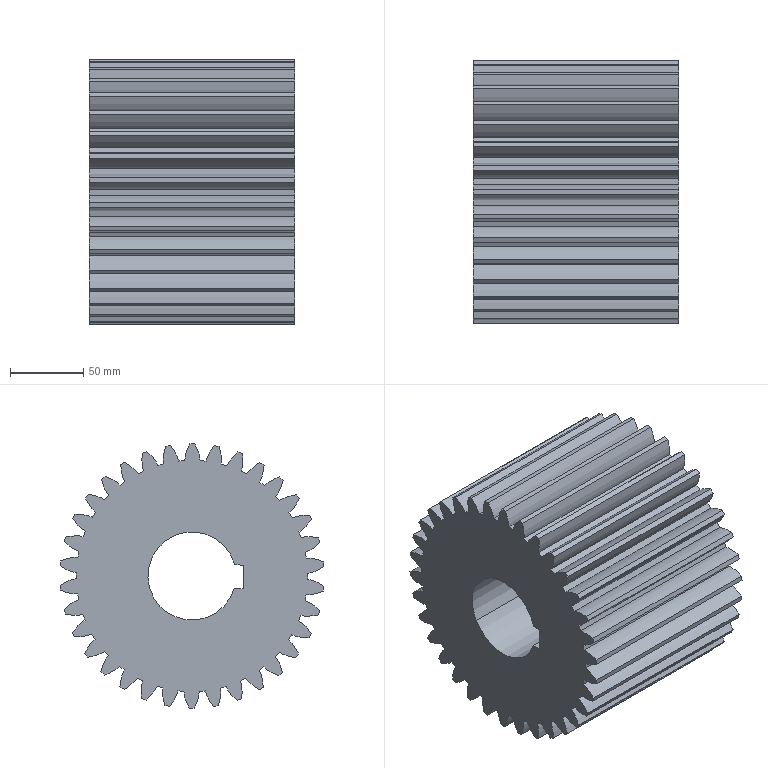Component | SolidWorks | Pinion-1 | 1 solid | 144 faces | box 140 x 179.55 x 179.98 mm | volume 2739604 mm3 | plane 73 | spline 68 | cylinder 3 | commonest cylinder face diameters 60 x3
build123d program:
from build123d import *

# Parameters (mm, degrees)
BOSS_EXTRUDE1_DEPTH           = 140
SKETCH1_R                     = 30
REPAIR_BORETOSHAFTDIA60_DEPTH = 71.5


with BuildPart() as part:
    # Sketch1_2 → Boss-Extrude1 (new body)
    with BuildSketch(Plane.XY.offset(140)):
        with BuildLine():
            Line((78.053, 10.453), (77.409, 14.47))
            add(Edge.make_bspline(
                [(77.409, 14.47), (82.062, 15.66), (87.574, 20.756)],
                knots=[3.749, 3.749, 3.749, 4.922, 4.922, 4.922], degree=2, weights=[1, 0.8327, 1]))
            Line((87.574, 20.756), (86.739, 24.006))
            add(Edge.make_bspline(
                [(86.739, 24.006), (79.432, 25.831), (74.803, 24.617)],
                knots=[1.318, 1.318, 1.318, 2.544, 2.544, 2.544], degree=2, weights=[1, 0.8179, 1]))
            Line((74.803, 24.617), (73.432, 28.448))
            add(Edge.make_bspline(
                [(73.432, 28.448), (77.787, 30.472), (82.269, 36.495)],
                knots=[0.607, 0.607, 0.607, 1.781, 1.781, 1.781], degree=2, weights=[1, 0.8327, 1]))
            Line((82.269, 36.495), (80.851, 39.536))
            add(Edge.make_bspline(
                [(80.851, 39.536), (73.333, 39.987), (69.006, 37.943)],
                knots=[1.318, 1.318, 1.318, 2.544, 2.544, 2.544], degree=2, weights=[1, 0.8179, 1]))
            Line((69.006, 37.943), (66.955, 41.457))
            add(Edge.make_bspline(
                [(66.955, 41.457), (70.864, 44.247), (74.162, 50.99)],
                knots=[0.607, 0.607, 0.607, 1.781, 1.781, 1.781], degree=2, weights=[1, 0.8327, 1]))
            Line((74.162, 50.99), (72.21, 53.719))
            add(Edge.make_bspline(
                [(72.21, 53.719), (64.737, 52.781), (60.859, 49.977)],
                knots=[1.318, 1.318, 1.318, 2.544, 2.544, 2.544], degree=2, weights=[1, 0.8179, 1]))
            Line((60.859, 49.977), (58.197, 53.054))
            add(Edge.make_bspline(
                [(58.197, 53.054), (61.527, 56.514), (63.53, 63.749)],
                knots=[0.607, 0.607, 0.607, 1.781, 1.781, 1.781], degree=2, weights=[1, 0.8327, 1]))
            Line((63.53, 63.749), (61.109, 66.073))
            add(Edge.make_bspline(
                [(61.109, 66.073), (53.936, 63.777), (50.64, 60.309)],
                knots=[1.318, 1.318, 1.318, 2.544, 2.544, 2.544], degree=2, weights=[1, 0.8179, 1]))
            Line((50.64, 60.309), (47.457, 62.844))
            add(Edge.make_bspline(
                [(47.457, 62.844), (50.095, 66.858), (50.734, 74.337)],
                knots=[3.749, 3.749, 3.749, 4.922, 4.922, 4.922], degree=2, weights=[1, 0.8327, 1]))
            Line((50.734, 74.337), (47.928, 76.177))
            add(Edge.make_bspline(
                [(47.928, 76.177), (41.299, 72.602), (38.696, 68.587)],
                knots=[1.318, 1.318, 1.318, 2.544, 2.544, 2.544], degree=2, weights=[1, 0.8179, 1]))
            Line((38.696, 68.587), (35.102, 70.494))
            add(Edge.make_bspline(
                [(35.102, 70.494), (36.957, 74.924), (36.211, 82.394)],
                knots=[0.607, 0.607, 0.607, 1.781, 1.781, 1.781], degree=2, weights=[1, 0.8327, 1]))
            Line((36.211, 82.394), (33.114, 83.687))
            add(Edge.make_bspline(
                [(33.114, 83.687), (27.255, 78.955), (25.434, 74.53)],
                knots=[1.318, 1.318, 1.318, 2.544, 2.544, 2.544], degree=2, weights=[1, 0.8179, 1]))
            Line((25.434, 74.53), (21.551, 75.744))
            add(Edge.make_bspline(
                [(21.551, 75.744), (22.56, 80.439), (20.455, 87.645)],
                knots=[0.607, 0.607, 0.607, 1.781, 1.781, 1.781], degree=2, weights=[1, 0.8327, 1]))
            Line((20.455, 87.645), (17.173, 88.346))
            add(Edge.make_bspline(
                [(17.173, 88.346), (12.283, 82.618), (11.306, 77.934)],
                knots=[4.459, 4.459, 4.459, 5.685, 5.685, 5.685], degree=2, weights=[1, 0.8179, 1]))
            Line((11.306, 77.934), (7.266, 78.414))
            add(Edge.make_bspline(
                [(7.266, 78.414), (7.395, 83.215), (4.002, 89.911)],
                knots=[0.607, 0.607, 0.607, 1.781, 1.781, 1.781], degree=2, weights=[1, 0.8327, 1]))
            Line((4.002, 89.911), (0.6472, 89.998))
            add(Edge.make_bspline(
                [(0.6472, 89.998), (-3.107, 83.469), (-3.207, 78.685)],
                knots=[4.459, 4.459, 4.459, 5.685, 5.685, 5.685], degree=2, weights=[1, 0.8179, 1]))
            Line((-3.207, 78.685), (-7.266, 78.414))
            add(Edge.make_bspline(
                [(-7.266, 78.414), (-8.021, 83.157), (-12.588, 89.115)],
                knots=[0.607, 0.607, 0.607, 1.781, 1.781, 1.781], degree=2, weights=[1, 0.8327, 1]))
            Line((-12.588, 89.115), (-15.901, 88.584))
            add(Edge.make_bspline(
                [(-15.901, 88.584), (-18.392, 81.476), (-17.61, 76.756)],
                knots=[4.459, 4.459, 4.459, 5.685, 5.685, 5.685], degree=2, weights=[1, 0.8179, 1]))
            Line((-17.61, 76.756), (-21.551, 75.744))
            add(Edge.make_bspline(
                [(-21.551, 75.744), (-23.165, 80.267), (-28.748, 85.285)],
                knots=[0.607, 0.607, 0.607, 1.781, 1.781, 1.781], degree=2, weights=[1, 0.8327, 1]))
            Line((-28.748, 85.285), (-31.907, 84.154))
            add(Edge.make_bspline(
                [(-31.907, 84.154), (-33.05, 76.71), (-31.414, 72.213)],
                knots=[4.459, 4.459, 4.459, 5.685, 5.685, 5.685], degree=2, weights=[1, 0.8179, 1]))
            Line((-31.414, 72.213), (-35.102, 70.494))
            add(Edge.make_bspline(
                [(-35.102, 70.494), (-37.519, 74.644), (-43.93, 78.55)],
                knots=[0.607, 0.607, 0.607, 1.781, 1.781, 1.781], degree=2, weights=[1, 0.8327, 1]))
            Line((-43.93, 78.55), (-46.827, 76.858))
            add(Edge.make_bspline(
                [(-46.827, 76.858), (-46.582, 69.331), (-44.149, 65.211)],
                knots=[4.459, 4.459, 4.459, 5.685, 5.685, 5.685], degree=2, weights=[1, 0.8179, 1]))
            Line((-44.149, 65.211), (-47.457, 62.844))
            add(Edge.make_bspline(
                [(-47.457, 62.844), (-50.596, 66.479), (-57.615, 69.141)],
                knots=[3.749, 3.749, 3.749, 4.922, 4.922, 4.922], degree=2, weights=[1, 0.8327, 1]))
            Line((-57.615, 69.141), (-60.153, 66.945))
            add(Edge.make_bspline(
                [(-60.153, 66.945), (-58.529, 59.591), (-55.379, 55.988)],
                knots=[4.459, 4.459, 4.459, 5.685, 5.685, 5.685], degree=2, weights=[1, 0.8179, 1]))
            Line((-55.379, 55.988), (-58.197, 53.054))
            add(Edge.make_bspline(
                [(-58.197, 53.054), (-61.95, 56.05), (-69.339, 57.377)],
                knots=[0.607, 0.607, 0.607, 1.781, 1.781, 1.781], degree=2, weights=[1, 0.8327, 1]))
            Line((-69.339, 57.377), (-71.43, 54.752))
            add(Edge.make_bspline(
                [(-71.43, 54.752), (-68.482, 47.821), (-64.724, 44.859)],
                knots=[1.318, 1.318, 1.318, 2.544, 2.544, 2.544], degree=2, weights=[1, 0.8179, 1]))
            Line((-64.724, 44.859), (-66.955, 41.457))
            add(Edge.make_bspline(
                [(-66.955, 41.457), (-71.194, 43.712), (-78.701, 43.659)],
                knots=[0.607, 0.607, 0.607, 1.781, 1.781, 1.781], degree=2, weights=[1, 0.8327, 1]))
            Line((-78.701, 43.659), (-80.274, 40.695))
            add(Edge.make_bspline(
                [(-80.274, 40.695), (-76.103, 34.424), (-71.865, 32.202)],
                knots=[4.459, 4.459, 4.459, 5.685, 5.685, 5.685], degree=2, weights=[1, 0.8179, 1]))
            Line((-71.865, 32.202), (-73.432, 28.448))
            add(Edge.make_bspline(
                [(-73.432, 28.448), (-78.014, 29.886), (-85.384, 28.454)],
                knots=[0.607, 0.607, 0.607, 1.781, 1.781, 1.781], degree=2, weights=[1, 0.8327, 1]))
            Line((-85.384, 28.454), (-86.385, 25.252))
            add(Edge.make_bspline(
                [(-86.385, 25.252), (-81.133, 19.854), (-76.559, 18.449)],
                knots=[4.459, 4.459, 4.459, 5.685, 5.685, 5.685], degree=2, weights=[1, 0.8179, 1]))
            Line((-76.559, 18.449), (-77.409, 14.47))
            add(Edge.make_bspline(
                [(-77.409, 14.47), (-82.178, 15.042), (-89.158, 12.28)],
                knots=[0.607, 0.607, 0.607, 1.781, 1.781, 1.781], degree=2, weights=[1, 0.8327, 1]))
            Line((-89.158, 12.28), (-89.554, 8.948))
            add(Edge.make_bspline(
                [(-89.554, 8.948), (-83.399, 4.608), (-78.645, 4.067)],
                knots=[4.459, 4.459, 4.459, 5.685, 5.685, 5.685], degree=2, weights=[1, 0.8179, 1]))
            Line((-78.645, 4.067), (-78.75, 0))
            add(Edge.make_bspline(
                [(-78.75, 0), (-83.542, -0.3143), (-89.897, -4.311)],
                knots=[3.749, 3.749, 3.749, 4.922, 4.922, 4.922], degree=2, weights=[1, 0.8327, 1]))
            Line((-89.897, -4.311), (-89.673, -7.659))
            add(Edge.make_bspline(
                [(-89.673, -7.659), (-82.826, -10.795), (-78.053, -10.453)],
                knots=[4.459, 4.459, 4.459, 5.685, 5.685, 5.685], degree=2, weights=[1, 0.8179, 1]))
            Line((-78.053, -10.453), (-77.409, -14.47))
            add(Edge.make_bspline(
                [(-77.409, -14.47), (-82.062, -15.66), (-87.574, -20.756)],
                knots=[0.607, 0.607, 0.607, 1.781, 1.781, 1.781], degree=2, weights=[1, 0.8327, 1]))
            Line((-87.574, -20.756), (-86.739, -24.006))
            add(Edge.make_bspline(
                [(-86.739, -24.006), (-79.432, -25.831), (-74.803, -24.617)],
                knots=[4.459, 4.459, 4.459, 5.685, 5.685, 5.685], degree=2, weights=[1, 0.8179, 1]))
            Line((-74.803, -24.617), (-73.432, -28.448))
            add(Edge.make_bspline(
                [(-73.432, -28.448), (-77.787, -30.472), (-82.269, -36.495)],
                knots=[3.749, 3.749, 3.749, 4.922, 4.922, 4.922], degree=2, weights=[1, 0.8327, 1]))
            Line((-82.269, -36.495), (-80.851, -39.536))
            add(Edge.make_bspline(
                [(-80.851, -39.536), (-73.333, -39.987), (-69.006, -37.943)],
                knots=[4.459, 4.459, 4.459, 5.685, 5.685, 5.685], degree=2, weights=[1, 0.8179, 1]))
            Line((-69.006, -37.943), (-66.955, -41.457))
            add(Edge.make_bspline(
                [(-66.955, -41.457), (-70.864, -44.247), (-74.162, -50.99)],
                knots=[3.749, 3.749, 3.749, 4.922, 4.922, 4.922], degree=2, weights=[1, 0.8327, 1]))
            Line((-74.162, -50.99), (-72.21, -53.719))
            add(Edge.make_bspline(
                [(-72.21, -53.719), (-64.737, -52.781), (-60.859, -49.977)],
                knots=[4.459, 4.459, 4.459, 5.685, 5.685, 5.685], degree=2, weights=[1, 0.8179, 1]))
            Line((-60.859, -49.977), (-58.197, -53.054))
            add(Edge.make_bspline(
                [(-58.197, -53.054), (-61.527, -56.514), (-63.53, -63.749)],
                knots=[3.749, 3.749, 3.749, 4.922, 4.922, 4.922], degree=2, weights=[1, 0.8327, 1]))
            Line((-63.53, -63.749), (-61.109, -66.073))
            add(Edge.make_bspline(
                [(-61.109, -66.073), (-53.936, -63.777), (-50.64, -60.309)],
                knots=[4.459, 4.459, 4.459, 5.685, 5.685, 5.685], degree=2, weights=[1, 0.8179, 1]))
            Line((-50.64, -60.309), (-47.457, -62.844))
            add(Edge.make_bspline(
                [(-47.457, -62.844), (-50.095, -66.858), (-50.734, -74.337)],
                knots=[3.749, 3.749, 3.749, 4.922, 4.922, 4.922], degree=2, weights=[1, 0.8327, 1]))
            Line((-50.734, -74.337), (-47.928, -76.177))
            add(Edge.make_bspline(
                [(-47.928, -76.177), (-41.299, -72.602), (-38.696, -68.587)],
                knots=[4.459, 4.459, 4.459, 5.685, 5.685, 5.685], degree=2, weights=[1, 0.8179, 1]))
            Line((-38.696, -68.587), (-35.102, -70.494))
            add(Edge.make_bspline(
                [(-35.102, -70.494), (-36.957, -74.924), (-36.211, -82.394)],
                knots=[3.749, 3.749, 3.749, 4.922, 4.922, 4.922], degree=2, weights=[1, 0.8327, 1]))
            Line((-36.211, -82.394), (-33.114, -83.687))
            add(Edge.make_bspline(
                [(-33.114, -83.687), (-27.255, -78.955), (-25.434, -74.53)],
                knots=[4.459, 4.459, 4.459, 5.685, 5.685, 5.685], degree=2, weights=[1, 0.8179, 1]))
            Line((-25.434, -74.53), (-21.551, -75.744))
            add(Edge.make_bspline(
                [(-21.551, -75.744), (-22.56, -80.439), (-20.455, -87.645)],
                knots=[3.749, 3.749, 3.749, 4.922, 4.922, 4.922], degree=2, weights=[1, 0.8327, 1]))
            Line((-20.455, -87.645), (-17.173, -88.346))
            add(Edge.make_bspline(
                [(-17.173, -88.346), (-12.283, -82.618), (-11.306, -77.934)],
                knots=[1.318, 1.318, 1.318, 2.544, 2.544, 2.544], degree=2, weights=[1, 0.8179, 1]))
            Line((-11.306, -77.934), (-7.266, -78.414))
            add(Edge.make_bspline(
                [(-7.266, -78.414), (-7.395, -83.215), (-4.002, -89.911)],
                knots=[3.749, 3.749, 3.749, 4.922, 4.922, 4.922], degree=2, weights=[1, 0.8327, 1]))
            Line((-4.002, -89.911), (-0.6472, -89.998))
            add(Edge.make_bspline(
                [(-0.6472, -89.998), (3.107, -83.469), (3.207, -78.685)],
                knots=[1.318, 1.318, 1.318, 2.544, 2.544, 2.544], degree=2, weights=[1, 0.8179, 1]))
            Line((3.207, -78.685), (7.266, -78.414))
            add(Edge.make_bspline(
                [(7.266, -78.414), (8.021, -83.157), (12.588, -89.115)],
                knots=[3.749, 3.749, 3.749, 4.922, 4.922, 4.922], degree=2, weights=[1, 0.8327, 1]))
            Line((12.588, -89.115), (15.901, -88.584))
            add(Edge.make_bspline(
                [(15.901, -88.584), (18.392, -81.476), (17.61, -76.756)],
                knots=[1.318, 1.318, 1.318, 2.544, 2.544, 2.544], degree=2, weights=[1, 0.8179, 1]))
            Line((17.61, -76.756), (21.551, -75.744))
            add(Edge.make_bspline(
                [(21.551, -75.744), (23.165, -80.267), (28.748, -85.285)],
                knots=[3.749, 3.749, 3.749, 4.922, 4.922, 4.922], degree=2, weights=[1, 0.8327, 1]))
            Line((28.748, -85.285), (31.907, -84.154))
            add(Edge.make_bspline(
                [(31.907, -84.154), (33.05, -76.71), (31.414, -72.213)],
                knots=[1.318, 1.318, 1.318, 2.544, 2.544, 2.544], degree=2, weights=[1, 0.8179, 1]))
            Line((31.414, -72.213), (35.102, -70.494))
            add(Edge.make_bspline(
                [(35.102, -70.494), (37.519, -74.644), (43.93, -78.55)],
                knots=[3.749, 3.749, 3.749, 4.922, 4.922, 4.922], degree=2, weights=[1, 0.8327, 1]))
            Line((43.93, -78.55), (46.827, -76.858))
            add(Edge.make_bspline(
                [(46.827, -76.858), (46.582, -69.331), (44.149, -65.211)],
                knots=[1.318, 1.318, 1.318, 2.544, 2.544, 2.544], degree=2, weights=[1, 0.8179, 1]))
            Line((44.149, -65.211), (47.457, -62.844))
            add(Edge.make_bspline(
                [(47.457, -62.844), (50.596, -66.479), (57.615, -69.141)],
                knots=[3.749, 3.749, 3.749, 4.922, 4.922, 4.922], degree=2, weights=[1, 0.8327, 1]))
            Line((57.615, -69.141), (60.153, -66.945))
            add(Edge.make_bspline(
                [(60.153, -66.945), (58.529, -59.591), (55.379, -55.988)],
                knots=[1.318, 1.318, 1.318, 2.544, 2.544, 2.544], degree=2, weights=[1, 0.8179, 1]))
            Line((55.379, -55.988), (58.197, -53.054))
            add(Edge.make_bspline(
                [(58.197, -53.054), (61.95, -56.05), (69.339, -57.377)],
                knots=[3.749, 3.749, 3.749, 4.922, 4.922, 4.922], degree=2, weights=[1, 0.8327, 1]))
            Line((69.339, -57.377), (71.43, -54.752))
            add(Edge.make_bspline(
                [(71.43, -54.752), (68.482, -47.821), (64.724, -44.859)],
                knots=[1.318, 1.318, 1.318, 2.544, 2.544, 2.544], degree=2, weights=[1, 0.8179, 1]))
            Line((64.724, -44.859), (66.955, -41.457))
            add(Edge.make_bspline(
                [(66.955, -41.457), (71.194, -43.712), (78.701, -43.659)],
                knots=[3.749, 3.749, 3.749, 4.922, 4.922, 4.922], degree=2, weights=[1, 0.8327, 1]))
            Line((78.701, -43.659), (80.274, -40.695))
            add(Edge.make_bspline(
                [(80.274, -40.695), (76.103, -34.424), (71.865, -32.202)],
                knots=[1.318, 1.318, 1.318, 2.544, 2.544, 2.544], degree=2, weights=[1, 0.8179, 1]))
            Line((71.865, -32.202), (73.432, -28.448))
            add(Edge.make_bspline(
                [(73.432, -28.448), (78.014, -29.886), (85.384, -28.454)],
                knots=[3.749, 3.749, 3.749, 4.922, 4.922, 4.922], degree=2, weights=[1, 0.8327, 1]))
            Line((85.384, -28.454), (86.385, -25.252))
            add(Edge.make_bspline(
                [(86.385, -25.252), (81.133, -19.854), (76.559, -18.449)],
                knots=[1.318, 1.318, 1.318, 2.544, 2.544, 2.544], degree=2, weights=[1, 0.8179, 1]))
            Line((76.559, -18.449), (77.409, -14.47))
            add(Edge.make_bspline(
                [(77.409, -14.47), (82.178, -15.042), (89.158, -12.28)],
                knots=[3.749, 3.749, 3.749, 4.922, 4.922, 4.922], degree=2, weights=[1, 0.8327, 1]))
            Line((89.158, -12.28), (89.554, -8.948))
            add(Edge.make_bspline(
                [(89.554, -8.948), (83.399, -4.608), (78.645, -4.067)],
                knots=[1.318, 1.318, 1.318, 2.544, 2.544, 2.544], degree=2, weights=[1, 0.8179, 1]))
            Line((78.645, -4.067), (78.75, 0))
            add(Edge.make_bspline(
                [(78.75, 0), (83.542, 0.3143), (89.897, 4.311)],
                knots=[3.749, 3.749, 3.749, 4.922, 4.922, 4.922], degree=2, weights=[1, 0.8327, 1]))
            Line((89.897, 4.311), (89.673, 7.659))
            add(Edge.make_bspline(
                [(89.673, 7.659), (82.826, 10.795), (78.053, 10.453)],
                knots=[1.318, 1.318, 1.318, 2.544, 2.544, 2.544], degree=2, weights=[1, 0.8179, 1]))
        make_face()
        with BuildLine():
            Line((-19.774, -21.213), (-25.867, -24.875))
            Line((-25.867, -24.875), (-34.107, -11.16))
            Line((-34.107, -11.16), (-28.014, -7.499))
            ThreePointArc((-28.014, -7.499), (24.858, 14.936), (-19.774, -21.213))
        make_face(mode=Mode.SUBTRACT)
    extrude(amount=-BOSS_EXTRUDE1_DEPTH)

    # Sketch1 → Repair_BoreToShaftDia60 (cut, symmetric)
    with BuildSketch(Plane.XY.offset(69.832)):
        Circle(SKETCH1_R)
    extrude(amount=REPAIR_BORETOSHAFTDIA60_DEPTH, both=True, mode=Mode.SUBTRACT)


solid = part.part

# Placed as in the assembly
solid = solid.moved(Location((-119.332, 1335.766, 1014.597), (59.906, 90, 0)))